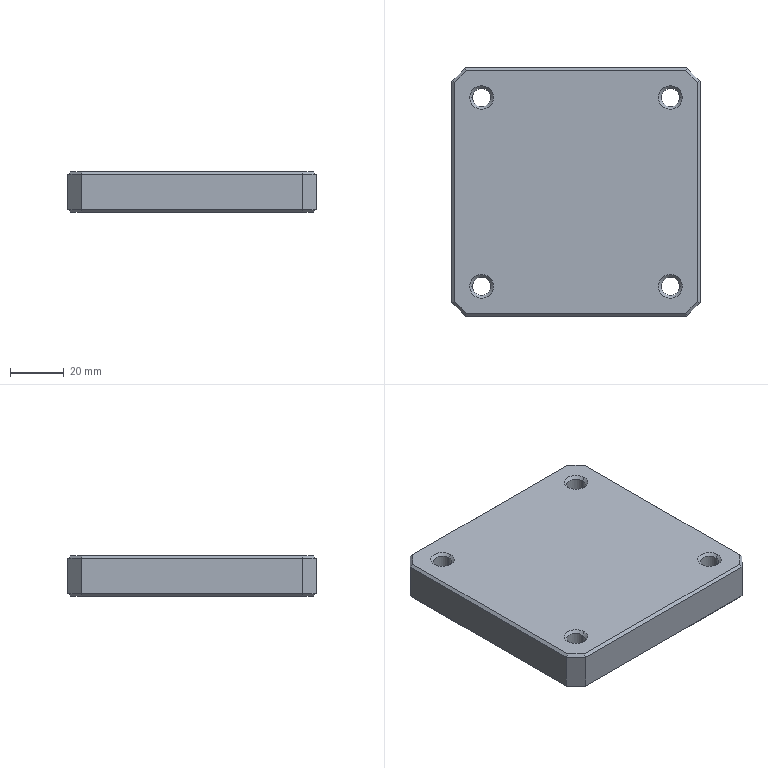Component | SolidWorks | 01-01FrameBody-1_03IntegratedCasterMount-1 | 1 solid | 50 faces | box 92 x 92 x 15 mm | volume 123583 mm3 | plane 26 | cone 16 | cylinder 8 | commonest cylinder face diameters 6.8 x8 | material 4040 Square Tube
build123d program:
from build123d import *

# Parameters (mm, degrees)
SKETCH1_W           = 92
SKETCH1_H           = 92
BOSS_EXTRUDE1_DEPTH = 15
M8_TAPPED_HOLE1_D   = 6.8
CHAMFER1_SIZE       = 5
CHAMFER2_SIZE       = 1


with BuildPart() as part:
    # Sketch1 → Boss-Extrude1 (new body)
    with BuildSketch(Plane(origin=(0, 0, 0), x_dir=(1, 0, 0), z_dir=(0, 1, 0))):
        Rectangle(SKETCH1_W, SKETCH1_H)
    extrude(amount=BOSS_EXTRUDE1_DEPTH)

    # M8 Tapped Hole1 (through all)
    with Locations(Plane(origin=(0, 15, 0), x_dir=(-1, 0, 0), z_dir=(0, 1, 0))):
        with Locations((35, 35), (35, -35), (-35, -35), (-35, 35)):
            Hole(M8_TAPPED_HOLE1_D / 2)

    # Chamfer1
    chamfer1_edges = [part.edges().sort_by_distance(p)[0] for p in [
        (-46, 7.5, -46),
        (46, 7.5, -46),
        (46, 7.5, 46),
        (-46, 7.5, 46),
    ]]
    chamfer(chamfer1_edges, length=CHAMFER1_SIZE)

    # Chamfer2
    chamfer2_edges = [part.edges().sort_by_distance(p)[0] for p in [
        (31.6, 15, 35),
        (31.6, 0, 35),
        (31.6, 15, -35),
        (31.6, 0, -35),
        (-38.4, 15, -35),
        (-38.4, 0, -35),
        (-38.4, 15, 35),
        (-38.4, 0, 35),
        (-46, 0, 0),
        (-46, 15, 0),
        (0, 0, -46),
        (46, 0, 0),
        (0, 0, 46),
        (-43.5, 0, 43.5),
        (43.5, 0, 43.5),
        (43.5, 0, -43.5),
        (-43.5, 0, -43.5),
        (0, 15, -46),
        (0, 15, 46),
        (46, 15, 0),
        (-43.5, 15, 43.5),
        (43.5, 15, 43.5),
        (43.5, 15, -43.5),
        (-43.5, 15, -43.5),
    ]]
    chamfer(chamfer2_edges, length=CHAMFER2_SIZE)


solid = part.part

# Placed as in the assembly
solid = solid.moved(Location((-46, 46, 0), (90, 0, 0)))